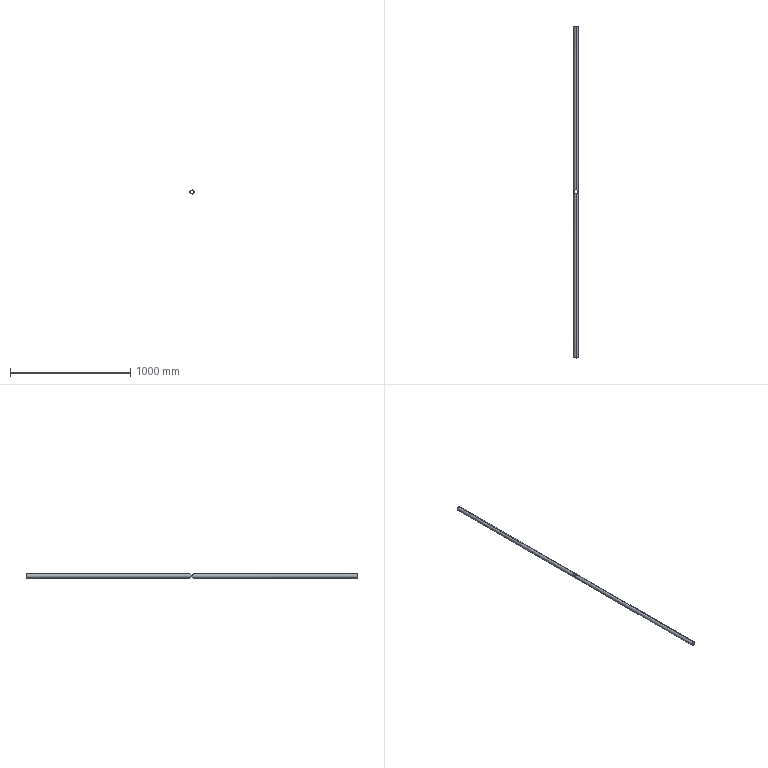Component | SolidWorks | PlatformGuardrail5-1 | 2 solids | 12 faces | box 33.5 x 2760 x 33.5 mm | volume 786282 mm3 | cylinder 10 | plane 2 | commonest cylinder face diameters 27.5 x4 33.5 x4 33.6 x2 | material Plain Carbon Steel
STEP:
#1=CARTESIAN_POINT('',(246.892,87.591,243.001));
#2=VERTEX_POINT('',#1);
#3=CARTESIAN_POINT('',(246.892,87.591,244.084));
#4=VERTEX_POINT('',#3);
#5=CARTESIAN_POINT('',(246.892,87.591,243.542));
#6=DIRECTION('',(0.,1.,0.));
#7=DIRECTION('',(0.,0.,1.));
#8=AXIS2_PLACEMENT_3D('',#5,#6,#7);
#9=CIRCLE('',#8,0.5413);
#10=EDGE_CURVE('',#2,#4,#9,.T.);
#11=ORIENTED_EDGE('',*,*,#10,.T.);
#12=CARTESIAN_POINT('',(246.892,34.05,244.084));
#13=VERTEX_POINT('',#12);
#14=CARTESIAN_POINT('',(246.892,87.591,244.084));
#15=DIRECTION('',(0.,-1.,0.));
#16=VECTOR('',#15,39.37);
#17=LINE('',#14,#16);
#18=EDGE_CURVE('',#4,#13,#17,.T.);
#19=ORIENTED_EDGE('',*,*,#18,.T.);
#20=CARTESIAN_POINT('',(246.892,34.05,243.001));
#21=VERTEX_POINT('',#20);
#22=CARTESIAN_POINT('',(246.892,34.05,243.001));
#23=CARTESIAN_POINT('',(246.854,34.05,243.001));
#24=CARTESIAN_POINT('',(246.816,34.047,243.005));
#25=CARTESIAN_POINT('',(246.762,34.038,243.016));
#26=CARTESIAN_POINT('',(246.744,34.034,243.021));
#27=CARTESIAN_POINT('',(246.709,34.025,243.032));
#28=CARTESIAN_POINT('',(246.692,34.019,243.039));
#29=CARTESIAN_POINT('',(246.659,34.008,243.053));
#30=CARTESIAN_POINT('',(246.643,34.002,243.061));
#31=CARTESIAN_POINT('',(246.612,33.988,243.078));
#32=CARTESIAN_POINT('',(246.597,33.981,243.088));
#33=CARTESIAN_POINT('',(246.555,33.959,243.117));
#34=CARTESIAN_POINT('',(246.529,33.942,243.139));
#35=CARTESIAN_POINT('',(246.494,33.917,243.175));
#36=CARTESIAN_POINT('',(246.482,33.908,243.188));
#37=CARTESIAN_POINT('',(246.461,33.891,243.214));
#38=CARTESIAN_POINT('',(246.451,33.882,243.227));
#39=CARTESIAN_POINT('',(246.423,33.856,243.269));
#40=CARTESIAN_POINT('',(246.407,33.839,243.298));
#41=CARTESIAN_POINT('',(246.387,33.816,243.346));
#42=CARTESIAN_POINT('',(246.381,33.809,243.362));
#43=CARTESIAN_POINT('',(246.37,33.796,243.396));
#44=CARTESIAN_POINT('',(246.366,33.79,243.413));
#45=CARTESIAN_POINT('',(246.358,33.78,243.449));
#46=CARTESIAN_POINT('',(246.355,33.776,243.467));
#47=CARTESIAN_POINT('',(246.351,33.77,243.505));
#48=CARTESIAN_POINT('',(246.35,33.769,243.524));
#49=CARTESIAN_POINT('',(246.35,33.769,243.561));
#50=CARTESIAN_POINT('',(246.351,33.77,243.58));
#51=CARTESIAN_POINT('',(246.354,33.774,243.608));
#52=CARTESIAN_POINT('',(246.356,33.776,243.617));
#53=CARTESIAN_POINT('',(246.358,33.78,243.636));
#54=CARTESIAN_POINT('',(246.36,33.782,243.645));
#55=CARTESIAN_POINT('',(246.366,33.79,243.671));
#56=CARTESIAN_POINT('',(246.37,33.796,243.689));
#57=CARTESIAN_POINT('',(246.381,33.809,243.722));
#58=CARTESIAN_POINT('',(246.387,33.816,243.739));
#59=CARTESIAN_POINT('',(246.407,33.84,243.787));
#60=CARTESIAN_POINT('',(246.423,33.857,243.816));
#61=CARTESIAN_POINT('',(246.451,33.882,243.858));
#62=CARTESIAN_POINT('',(246.461,33.891,243.871));
#63=CARTESIAN_POINT('',(246.483,33.908,243.897));
#64=CARTESIAN_POINT('',(246.494,33.917,243.91));
#65=CARTESIAN_POINT('',(246.529,33.943,243.946));
#66=CARTESIAN_POINT('',(246.555,33.959,243.967));
#67=CARTESIAN_POINT('',(246.597,33.981,243.997));
#68=CARTESIAN_POINT('',(246.612,33.988,244.006));
#69=CARTESIAN_POINT('',(246.643,34.002,244.023));
#70=CARTESIAN_POINT('',(246.659,34.008,244.031));
#71=CARTESIAN_POINT('',(246.692,34.02,244.046));
#72=CARTESIAN_POINT('',(246.709,34.025,244.052));
#73=CARTESIAN_POINT('',(246.744,34.034,244.063));
#74=CARTESIAN_POINT('',(246.762,34.037,244.068));
#75=CARTESIAN_POINT('',(246.817,34.047,244.08));
#76=CARTESIAN_POINT('',(246.854,34.05,244.084));
#77=CARTESIAN_POINT('',(246.892,34.05,244.084));
#78=B_SPLINE_CURVE_WITH_KNOTS('',3,(#22,#23,#24,#25,#26,#27,#28,#29,#30,#31,#32,#33,#34,#35,#36,#37,#38,#39,#40,#41,#42,#43,#44,#45,#46,#47,#48,#49,#50,#51,#52,#53,#54,#55,#56,#57,#58,#59,#60,#61,#62,#63,#64,#65,#66,#67,#68,#69,#70,#71,#72,#73,#74,#75,#76,#77),.UNSPECIFIED.,.F.,.F.,(4,2,2,2,2,2,2,2,2,2,2,2,2,2,2,2,2,2,2,2,2,2,2,2,2,2,2,4),(0.,0.002859,0.004288,0.005717,0.007146,0.008576,0.01143,0.01286,0.01429,0.01715,0.01858,0.02001,0.02144,0.02287,0.0243,0.02501,0.02573,0.02716,0.02859,0.03144,0.03287,0.0343,0.03716,0.03859,0.04002,0.04145,0.04288,0.04574),.UNSPECIFIED.);
#79=EDGE_CURVE('',#21,#13,#78,.T.);
#80=ORIENTED_EDGE('',*,*,#79,.F.);
#81=CARTESIAN_POINT('',(246.892,87.591,243.001));
#82=DIRECTION('',(0.,-1.,0.));
#83=VECTOR('',#82,39.37);
#84=LINE('',#81,#83);
#85=EDGE_CURVE('',#2,#21,#84,.T.);
#86=ORIENTED_EDGE('',*,*,#85,.F.);
#87=EDGE_LOOP('',(#11,#19,#80,#86));
#88=FACE_OUTER_BOUND('',#87,.T.);
#89=CARTESIAN_POINT('',(246.892,87.591,243.542));
#90=DIRECTION('',(0.,-1.,0.));
#91=DIRECTION('',(0.,0.,-1.));
#92=AXIS2_PLACEMENT_3D('',#89,#90,#91);
#93=CYLINDRICAL_SURFACE('',#92,0.5413);
#94=ADVANCED_FACE('',(#88),#93,.F.);
#95=CARTESIAN_POINT('',(246.892,87.591,244.202));
#96=VERTEX_POINT('',#95);
#97=CARTESIAN_POINT('',(246.892,87.591,242.883));
#98=VERTEX_POINT('',#97);
#99=CARTESIAN_POINT('',(246.892,87.591,243.542));
#100=DIRECTION('',(0.,1.,0.));
#101=DIRECTION('',(0.,0.,1.));
#102=AXIS2_PLACEMENT_3D('',#99,#100,#101);
#103=CIRCLE('',#102,0.6594);
#104=EDGE_CURVE('',#96,#98,#103,.T.);
#105=ORIENTED_EDGE('',*,*,#104,.F.);
#106=CARTESIAN_POINT('',(246.892,34.05,244.202));
#107=VERTEX_POINT('',#106);
#108=CARTESIAN_POINT('',(246.892,87.591,244.202));
#109=DIRECTION('',(0.,-1.,0.));
#110=VECTOR('',#109,39.37);
#111=LINE('',#108,#110);
#112=EDGE_CURVE('',#96,#107,#111,.T.);
#113=ORIENTED_EDGE('',*,*,#112,.T.);
#114=CARTESIAN_POINT('',(246.892,34.05,242.883));
#115=VERTEX_POINT('',#114);
#116=CARTESIAN_POINT('',(246.892,34.05,244.202));
#117=CARTESIAN_POINT('',(246.918,34.05,244.202));
#118=CARTESIAN_POINT('',(246.943,34.049,244.2));
#119=CARTESIAN_POINT('',(246.981,34.044,244.196));
#120=CARTESIAN_POINT('',(246.994,34.042,244.194));
#121=CARTESIAN_POINT('',(247.019,34.038,244.189));
#122=CARTESIAN_POINT('',(247.031,34.035,244.187));
#123=CARTESIAN_POINT('',(247.068,34.027,244.178));
#124=CARTESIAN_POINT('',(247.092,34.02,244.171));
#125=CARTESIAN_POINT('',(247.126,34.007,244.159));
#126=CARTESIAN_POINT('',(247.138,34.003,244.154));
#127=CARTESIAN_POINT('',(247.16,33.993,244.145));
#128=CARTESIAN_POINT('',(247.171,33.988,244.14));
#129=CARTESIAN_POINT('',(247.224,33.962,244.114));
#130=CARTESIAN_POINT('',(247.262,33.938,244.09));
#131=CARTESIAN_POINT('',(247.314,33.898,244.049));
#132=CARTESIAN_POINT('',(247.331,33.884,244.035));
#133=CARTESIAN_POINT('',(247.362,33.855,244.006));
#134=CARTESIAN_POINT('',(247.376,33.84,243.99));
#135=CARTESIAN_POINT('',(247.416,33.794,243.944));
#136=CARTESIAN_POINT('',(247.439,33.762,243.912));
#137=CARTESIAN_POINT('',(247.469,33.712,243.861));
#138=CARTESIAN_POINT('',(247.478,33.695,243.844));
#139=CARTESIAN_POINT('',(247.495,33.66,243.809));
#140=CARTESIAN_POINT('',(247.503,33.643,243.792));
#141=CARTESIAN_POINT('',(247.516,33.609,243.756));
#142=CARTESIAN_POINT('',(247.522,33.591,243.738));
#143=CARTESIAN_POINT('',(247.532,33.556,243.702));
#144=CARTESIAN_POINT('',(247.536,33.539,243.684));
#145=CARTESIAN_POINT('',(247.541,33.513,243.656));
#146=CARTESIAN_POINT('',(247.543,33.504,243.646));
#147=CARTESIAN_POINT('',(247.546,33.488,243.627));
#148=CARTESIAN_POINT('',(247.547,33.479,243.617));
#149=CARTESIAN_POINT('',(247.549,33.467,243.602));
#150=CARTESIAN_POINT('',(247.549,33.463,243.597));
#151=CARTESIAN_POINT('',(247.55,33.456,243.586));
#152=CARTESIAN_POINT('',(247.55,33.452,243.581));
#153=CARTESIAN_POINT('',(247.551,33.446,243.569));
#154=CARTESIAN_POINT('',(247.551,33.444,243.564));
#155=CARTESIAN_POINT('',(247.551,33.44,243.551));
#156=CARTESIAN_POINT('',(247.551,33.439,243.545));
#157=CARTESIAN_POINT('',(247.551,33.44,243.532));
#158=CARTESIAN_POINT('',(247.551,33.442,243.525));
#159=CARTESIAN_POINT('',(247.551,33.447,243.513));
#160=CARTESIAN_POINT('',(247.55,33.45,243.508));
#161=CARTESIAN_POINT('',(247.549,33.46,243.491));
#162=CARTESIAN_POINT('',(247.548,33.468,243.481));
#163=CARTESIAN_POINT('',(247.546,33.484,243.461));
#164=CARTESIAN_POINT('',(247.545,33.493,243.452));
#165=CARTESIAN_POINT('',(247.542,33.509,243.433));
#166=CARTESIAN_POINT('',(247.54,33.518,243.423));
#167=CARTESIAN_POINT('',(247.535,33.544,243.396));
#168=CARTESIAN_POINT('',(247.531,33.561,243.377));
#169=CARTESIAN_POINT('',(247.52,33.596,243.341));
#170=CARTESIAN_POINT('',(247.514,33.613,243.323));
#171=CARTESIAN_POINT('',(247.494,33.665,243.271));
#172=CARTESIAN_POINT('',(247.477,33.699,243.236));
#173=CARTESIAN_POINT('',(247.438,33.764,243.17));
#174=CARTESIAN_POINT('',(247.415,33.796,243.138));
#175=CARTESIAN_POINT('',(247.374,33.842,243.092));
#176=CARTESIAN_POINT('',(247.359,33.857,243.077));
#177=CARTESIAN_POINT('',(247.329,33.886,243.048));
#178=CARTESIAN_POINT('',(247.312,33.9,243.034));
#179=CARTESIAN_POINT('',(247.278,33.926,243.007));
#180=CARTESIAN_POINT('',(247.26,33.939,242.995));
#181=CARTESIAN_POINT('',(247.221,33.963,242.971));
#182=CARTESIAN_POINT('',(247.201,33.974,242.959));
#183=CARTESIAN_POINT('',(247.159,33.994,242.939));
#184=CARTESIAN_POINT('',(247.137,34.004,242.929));
#185=CARTESIAN_POINT('',(247.102,34.016,242.917));
#186=CARTESIAN_POINT('',(247.091,34.02,242.913));
#187=CARTESIAN_POINT('',(247.067,34.027,242.906));
#188=CARTESIAN_POINT('',(247.055,34.03,242.903));
#189=CARTESIAN_POINT('',(247.018,34.038,242.895));
#190=CARTESIAN_POINT('',(246.993,34.043,242.89));
#191=CARTESIAN_POINT('',(246.956,34.047,242.886));
#192=CARTESIAN_POINT('',(246.943,34.048,242.885));
#193=CARTESIAN_POINT('',(246.924,34.049,242.884));
#194=CARTESIAN_POINT('',(246.918,34.05,242.883));
#195=CARTESIAN_POINT('',(246.905,34.05,242.883));
#196=CARTESIAN_POINT('',(246.898,34.05,242.883));
#197=CARTESIAN_POINT('',(246.892,34.05,242.883));
#198=B_SPLINE_CURVE_WITH_KNOTS('',3,(#116,#117,#118,#119,#120,#121,#122,#123,#124,#125,#126,#127,#128,#129,#130,#131,#132,#133,#134,#135,#136,#137,#138,#139,#140,#141,#142,#143,#144,#145,#146,#147,#148,#149,#150,#151,#152,#153,#154,#155,#156,#157,#158,#159,#160,#161,#162,#163,#164,#165,#166,#167,#168,#169,#170,#171,#172,#173,#174,#175,#176,#177,#178,#179,#180,#181,#182,#183,#184,#185,#186,#187,#188,#189,#190,#191,#192,#193,#194,#195,#196,#197),.UNSPECIFIED.,.F.,.F.,(4,2,2,2,2,2,2,2,2,2,2,2,2,2,2,2,2,2,2,2,2,2,2,2,2,2,2,2,2,2,2,2,2,2,2,2,2,2,2,2,4),(0.06181,0.06373,0.0647,0.06566,0.06759,0.06855,0.06951,0.07337,0.07529,0.07722,0.08107,0.083,0.08492,0.08685,0.08878,0.08974,0.0907,0.09118,0.09167,0.09215,0.09263,0.09311,0.09359,0.09456,0.09552,0.09648,0.09841,0.1003,0.1042,0.108,0.11,0.1119,0.1138,0.1157,0.1177,0.1186,0.1196,0.1215,0.1225,0.123,0.1235),.UNSPECIFIED.);
#199=EDGE_CURVE('',#107,#115,#198,.T.);
#200=ORIENTED_EDGE('',*,*,#199,.T.);
#201=CARTESIAN_POINT('',(246.892,87.591,242.883));
#202=DIRECTION('',(0.,-1.,0.));
#203=VECTOR('',#202,39.37);
#204=LINE('',#201,#203);
#205=EDGE_CURVE('',#98,#115,#204,.T.);
#206=ORIENTED_EDGE('',*,*,#205,.F.);
#207=EDGE_LOOP('',(#105,#113,#200,#206));
#208=FACE_OUTER_BOUND('',#207,.T.);
#209=CARTESIAN_POINT('',(246.892,87.591,243.542));
#210=DIRECTION('',(0.,-1.,0.));
#211=DIRECTION('',(0.,0.,-1.));
#212=AXIS2_PLACEMENT_3D('',#209,#210,#211);
#213=CYLINDRICAL_SURFACE('',#212,0.6594);
#214=ADVANCED_FACE('',(#208),#213,.T.);
#215=ORIENTED_EDGE('',*,*,#112,.F.);
#216=CARTESIAN_POINT('',(246.892,87.591,243.542));
#217=DIRECTION('',(0.,1.,0.));
#218=DIRECTION('',(0.,0.,1.));
#219=AXIS2_PLACEMENT_3D('',#216,#217,#218);
#220=CIRCLE('',#219,0.6594);
#221=EDGE_CURVE('',#98,#96,#220,.T.);
#222=ORIENTED_EDGE('',*,*,#221,.F.);
#223=ORIENTED_EDGE('',*,*,#205,.T.);
#224=CARTESIAN_POINT('',(246.892,34.05,242.883));
#225=CARTESIAN_POINT('',(246.84,34.05,242.883));
#226=CARTESIAN_POINT('',(246.79,34.044,242.889));
#227=CARTESIAN_POINT('',(246.729,34.03,242.903));
#228=CARTESIAN_POINT('',(246.717,34.027,242.906));
#229=CARTESIAN_POINT('',(246.694,34.02,242.913));
#230=CARTESIAN_POINT('',(246.682,34.016,242.917));
#231=CARTESIAN_POINT('',(246.648,34.004,242.929));
#232=CARTESIAN_POINT('',(246.626,33.995,242.938));
#233=CARTESIAN_POINT('',(246.584,33.975,242.959));
#234=CARTESIAN_POINT('',(246.563,33.963,242.97));
#235=CARTESIAN_POINT('',(246.525,33.94,242.994));
#236=CARTESIAN_POINT('',(246.507,33.927,243.006));
#237=CARTESIAN_POINT('',(246.473,33.901,243.033));
#238=CARTESIAN_POINT('',(246.456,33.887,243.047));
#239=CARTESIAN_POINT('',(246.426,33.858,243.075));
#240=CARTESIAN_POINT('',(246.411,33.844,243.09));
#241=CARTESIAN_POINT('',(246.37,33.798,243.136));
#242=CARTESIAN_POINT('',(246.347,33.766,243.168));
#243=CARTESIAN_POINT('',(246.307,33.701,243.234));
#244=CARTESIAN_POINT('',(246.291,33.667,243.268));
#245=CARTESIAN_POINT('',(246.27,33.616,243.321));
#246=CARTESIAN_POINT('',(246.264,33.598,243.339));
#247=CARTESIAN_POINT('',(246.254,33.564,243.375));
#248=CARTESIAN_POINT('',(246.249,33.546,243.393));
#249=CARTESIAN_POINT('',(246.243,33.52,243.421));
#250=CARTESIAN_POINT('',(246.242,33.512,243.43));
#251=CARTESIAN_POINT('',(246.239,33.495,243.449));
#252=CARTESIAN_POINT('',(246.238,33.486,243.459));
#253=CARTESIAN_POINT('',(246.235,33.47,243.478));
#254=CARTESIAN_POINT('',(246.234,33.462,243.488));
#255=CARTESIAN_POINT('',(246.233,33.452,243.504));
#256=CARTESIAN_POINT('',(246.233,33.449,243.51));
#257=CARTESIAN_POINT('',(246.233,33.443,243.522));
#258=CARTESIAN_POINT('',(246.232,33.441,243.528));
#259=CARTESIAN_POINT('',(246.232,33.439,243.541));
#260=CARTESIAN_POINT('',(246.232,33.44,243.547));
#261=CARTESIAN_POINT('',(246.233,33.442,243.56));
#262=CARTESIAN_POINT('',(246.233,33.445,243.566));
#263=CARTESIAN_POINT('',(246.234,33.454,243.584));
#264=CARTESIAN_POINT('',(246.234,33.461,243.594));
#265=CARTESIAN_POINT('',(246.236,33.477,243.615));
#266=CARTESIAN_POINT('',(246.237,33.485,243.624));
#267=CARTESIAN_POINT('',(246.24,33.502,243.644));
#268=CARTESIAN_POINT('',(246.242,33.511,243.653));
#269=CARTESIAN_POINT('',(246.247,33.537,243.682));
#270=CARTESIAN_POINT('',(246.251,33.554,243.7));
#271=CARTESIAN_POINT('',(246.261,33.59,243.737));
#272=CARTESIAN_POINT('',(246.267,33.607,243.755));
#273=CARTESIAN_POINT('',(246.287,33.659,243.808));
#274=CARTESIAN_POINT('',(246.303,33.693,243.843));
#275=CARTESIAN_POINT('',(246.333,33.743,243.893));
#276=CARTESIAN_POINT('',(246.344,33.76,243.91));
#277=CARTESIAN_POINT('',(246.367,33.792,243.942));
#278=CARTESIAN_POINT('',(246.38,33.808,243.958));
#279=CARTESIAN_POINT('',(246.42,33.854,244.005));
#280=CARTESIAN_POINT('',(246.451,33.884,244.035));
#281=CARTESIAN_POINT('',(246.503,33.924,244.075));
#282=CARTESIAN_POINT('',(246.521,33.937,244.088));
#283=CARTESIAN_POINT('',(246.56,33.961,244.113));
#284=CARTESIAN_POINT('',(246.58,33.973,244.124));
#285=CARTESIAN_POINT('',(246.623,33.993,244.145));
#286=CARTESIAN_POINT('',(246.645,34.003,244.154));
#287=CARTESIAN_POINT('',(246.691,34.019,244.171));
#288=CARTESIAN_POINT('',(246.715,34.027,244.178));
#289=CARTESIAN_POINT('',(246.764,34.038,244.19));
#290=CARTESIAN_POINT('',(246.789,34.043,244.194));
#291=CARTESIAN_POINT('',(246.84,34.049,244.2));
#292=CARTESIAN_POINT('',(246.866,34.05,244.202));
#293=CARTESIAN_POINT('',(246.892,34.05,244.202));
#294=B_SPLINE_CURVE_WITH_KNOTS('',3,(#224,#225,#226,#227,#228,#229,#230,#231,#232,#233,#234,#235,#236,#237,#238,#239,#240,#241,#242,#243,#244,#245,#246,#247,#248,#249,#250,#251,#252,#253,#254,#255,#256,#257,#258,#259,#260,#261,#262,#263,#264,#265,#266,#267,#268,#269,#270,#271,#272,#273,#274,#275,#276,#277,#278,#279,#280,#281,#282,#283,#284,#285,#286,#287,#288,#289,#290,#291,#292,#293),.UNSPECIFIED.,.F.,.F.,(4,2,2,2,2,2,2,2,2,2,2,2,2,2,2,2,2,2,2,2,2,2,2,2,2,2,2,2,2,2,2,2,2,2,4),(0.,0.003863,0.004829,0.005795,0.007726,0.009658,0.01159,0.01352,0.01545,0.01932,0.02318,0.02511,0.02704,0.02801,0.02897,0.02994,0.03042,0.0309,0.03139,0.03187,0.03284,0.0338,0.03477,0.0367,0.03863,0.04249,0.04442,0.04636,0.05022,0.05215,0.05408,0.05601,0.05795,0.05988,0.06181),.UNSPECIFIED.);
#295=EDGE_CURVE('',#115,#107,#294,.T.);
#296=ORIENTED_EDGE('',*,*,#295,.T.);
#297=EDGE_LOOP('',(#215,#222,#223,#296));
#298=FACE_OUTER_BOUND('',#297,.T.);
#299=CARTESIAN_POINT('',(246.892,87.591,243.542));
#300=DIRECTION('',(0.,-1.,0.));
#301=DIRECTION('',(0.,0.,-1.));
#302=AXIS2_PLACEMENT_3D('',#299,#300,#301);
#303=CYLINDRICAL_SURFACE('',#302,0.6594);
#304=ADVANCED_FACE('',(#298),#303,.T.);
#305=ORIENTED_EDGE('',*,*,#18,.F.);
#306=CARTESIAN_POINT('',(246.892,87.591,243.542));
#307=DIRECTION('',(0.,1.,0.));
#308=DIRECTION('',(0.,0.,1.));
#309=AXIS2_PLACEMENT_3D('',#306,#307,#308);
#310=CIRCLE('',#309,0.5413);
#311=EDGE_CURVE('',#4,#2,#310,.T.);
#312=ORIENTED_EDGE('',*,*,#311,.T.);
#313=ORIENTED_EDGE('',*,*,#85,.T.);
#314=CARTESIAN_POINT('',(246.892,34.05,244.084));
#315=CARTESIAN_POINT('',(246.901,34.05,244.084));
#316=CARTESIAN_POINT('',(246.911,34.05,244.083));
#317=CARTESIAN_POINT('',(246.929,34.049,244.082));
#318=CARTESIAN_POINT('',(246.939,34.048,244.082));
#319=CARTESIAN_POINT('',(246.967,34.046,244.079));
#320=CARTESIAN_POINT('',(246.986,34.044,244.076));
#321=CARTESIAN_POINT('',(247.022,34.037,244.068));
#322=CARTESIAN_POINT('',(247.04,34.034,244.063));
#323=CARTESIAN_POINT('',(247.075,34.025,244.052));
#324=CARTESIAN_POINT('',(247.092,34.019,244.046));
#325=CARTESIAN_POINT('',(247.125,34.008,244.031));
#326=CARTESIAN_POINT('',(247.141,34.002,244.023));
#327=CARTESIAN_POINT('',(247.171,33.988,244.006));
#328=CARTESIAN_POINT('',(247.186,33.981,243.997));
#329=CARTESIAN_POINT('',(247.229,33.959,243.967));
#330=CARTESIAN_POINT('',(247.255,33.942,243.945));
#331=CARTESIAN_POINT('',(247.29,33.917,243.909));
#332=CARTESIAN_POINT('',(247.301,33.908,243.897));
#333=CARTESIAN_POINT('',(247.322,33.891,243.871));
#334=CARTESIAN_POINT('',(247.332,33.882,243.858));
#335=CARTESIAN_POINT('',(247.36,33.856,243.816));
#336=CARTESIAN_POINT('',(247.376,33.84,243.786));
#337=CARTESIAN_POINT('',(247.396,33.817,243.739));
#338=CARTESIAN_POINT('',(247.402,33.809,243.723));
#339=CARTESIAN_POINT('',(247.413,33.796,243.69));
#340=CARTESIAN_POINT('',(247.418,33.79,243.672));
#341=CARTESIAN_POINT('',(247.425,33.78,243.636));
#342=CARTESIAN_POINT('',(247.428,33.776,243.618));
#343=CARTESIAN_POINT('',(247.431,33.772,243.59));
#344=CARTESIAN_POINT('',(247.432,33.771,243.581));
#345=CARTESIAN_POINT('',(247.433,33.769,243.562));
#346=CARTESIAN_POINT('',(247.433,33.769,243.552));
#347=CARTESIAN_POINT('',(247.433,33.769,243.524));
#348=CARTESIAN_POINT('',(247.432,33.77,243.505));
#349=CARTESIAN_POINT('',(247.428,33.775,243.468));
#350=CARTESIAN_POINT('',(247.425,33.78,243.45));
#351=CARTESIAN_POINT('',(247.414,33.795,243.396));
#352=CARTESIAN_POINT('',(247.404,33.808,243.362));
#353=CARTESIAN_POINT('',(247.383,33.831,243.315));
#354=CARTESIAN_POINT('',(247.376,33.84,243.299));
#355=CARTESIAN_POINT('',(247.36,33.856,243.269));
#356=CARTESIAN_POINT('',(247.351,33.865,243.255));
#357=CARTESIAN_POINT('',(247.323,33.891,243.214));
#358=CARTESIAN_POINT('',(247.302,33.908,243.188));
#359=CARTESIAN_POINT('',(247.267,33.934,243.151));
#360=CARTESIAN_POINT('',(247.254,33.942,243.14));
#361=CARTESIAN_POINT('',(247.228,33.958,243.118));
#362=CARTESIAN_POINT('',(247.215,33.966,243.108));
#363=CARTESIAN_POINT('',(247.173,33.988,243.078));
#364=CARTESIAN_POINT('',(247.142,34.002,243.061));
#365=CARTESIAN_POINT('',(247.093,34.019,243.039));
#366=CARTESIAN_POINT('',(247.075,34.024,243.033));
#367=CARTESIAN_POINT('',(247.041,34.033,243.021));
#368=CARTESIAN_POINT('',(247.023,34.037,243.017));
#369=CARTESIAN_POINT('',(246.986,34.044,243.009));
#370=CARTESIAN_POINT('',(246.968,34.046,243.006));
#371=CARTESIAN_POINT('',(246.93,34.049,243.002));
#372=CARTESIAN_POINT('',(246.911,34.05,243.001));
#373=CARTESIAN_POINT('',(246.892,34.05,243.001));
#374=B_SPLINE_CURVE_WITH_KNOTS('',3,(#314,#315,#316,#317,#318,#319,#320,#321,#322,#323,#324,#325,#326,#327,#328,#329,#330,#331,#332,#333,#334,#335,#336,#337,#338,#339,#340,#341,#342,#343,#344,#345,#346,#347,#348,#349,#350,#351,#352,#353,#354,#355,#356,#357,#358,#359,#360,#361,#362,#363,#364,#365,#366,#367,#368,#369,#370,#371,#372,#373),.UNSPECIFIED.,.F.,.F.,(4,2,2,2,2,2,2,2,2,2,2,2,2,2,2,2,2,2,2,2,2,2,2,2,2,2,2,2,2,4),(0.04574,0.04645,0.04716,0.04859,0.05001,0.05144,0.05286,0.05429,0.05714,0.05857,0.05999,0.06284,0.06427,0.0657,0.06712,0.06783,0.06855,0.06997,0.0714,0.07425,0.07568,0.0771,0.07995,0.08138,0.0828,0.08566,0.08708,0.08851,0.08993,0.09136),.UNSPECIFIED.);
#375=EDGE_CURVE('',#13,#21,#374,.T.);
#376=ORIENTED_EDGE('',*,*,#375,.F.);
#377=EDGE_LOOP('',(#305,#312,#313,#376));
#378=FACE_OUTER_BOUND('',#377,.T.);
#379=CARTESIAN_POINT('',(246.892,87.591,243.542));
#380=DIRECTION('',(0.,-1.,0.));
#381=DIRECTION('',(0.,0.,-1.));
#382=AXIS2_PLACEMENT_3D('',#379,#380,#381);
#383=CYLINDRICAL_SURFACE('',#382,0.5413);
#384=ADVANCED_FACE('',(#378),#383,.F.);
#385=ORIENTED_EDGE('',*,*,#221,.T.);
#386=ORIENTED_EDGE('',*,*,#104,.T.);
#387=EDGE_LOOP('',(#385,#386));
#388=FACE_OUTER_BOUND('',#387,.T.);
#389=ORIENTED_EDGE('',*,*,#10,.F.);
#390=ORIENTED_EDGE('',*,*,#311,.F.);
#391=EDGE_LOOP('',(#389,#390));
#392=FACE_BOUND('',#391,.T.);
#393=CARTESIAN_POINT('',(246.892,87.591,243.542));
#394=DIRECTION('',(0.,1.,0.));
#395=DIRECTION('',(0.,0.,1.));
#396=AXIS2_PLACEMENT_3D('',#393,#394,#395);
#397=PLANE('',#396);
#398=ADVANCED_FACE('',(#388,#392),#397,.T.);
#399=ORIENTED_EDGE('',*,*,#79,.T.);
#400=ORIENTED_EDGE('',*,*,#375,.T.);
#401=EDGE_LOOP('',(#399,#400));
#402=FACE_BOUND('',#401,.T.);
#403=ORIENTED_EDGE('',*,*,#295,.F.);
#404=ORIENTED_EDGE('',*,*,#199,.F.);
#405=EDGE_LOOP('',(#403,#404));
#406=FACE_OUTER_BOUND('',#405,.T.);
#407=CARTESIAN_POINT('',(246.892,33.389,242.883));
#408=DIRECTION('',(0.,0.,1.));
#409=DIRECTION('',(1.,0.,0.));
#410=AXIS2_PLACEMENT_3D('',#407,#408,#409);
#411=CYLINDRICAL_SURFACE('',#410,0.6614);
#412=ADVANCED_FACE('',(#402,#406),#411,.F.);
#413=CLOSED_SHELL('',(#94,#214,#304,#384,#398,#412));
#414=MANIFOLD_SOLID_BREP('',#413);
#415=CARTESIAN_POINT('',(246.892,32.727,244.084));
#416=VERTEX_POINT('',#415);
#417=CARTESIAN_POINT('',(246.892,32.727,243.001));
#418=VERTEX_POINT('',#417);
#419=CARTESIAN_POINT('',(246.892,32.727,244.084));
#420=CARTESIAN_POINT('',(246.882,32.727,244.084));
#421=CARTESIAN_POINT('',(246.873,32.727,244.083));
#422=CARTESIAN_POINT('',(246.854,32.728,244.082));
#423=CARTESIAN_POINT('',(246.845,32.729,244.082));
#424=CARTESIAN_POINT('',(246.816,32.731,244.079));
#425=CARTESIAN_POINT('',(246.798,32.734,244.076));
#426=CARTESIAN_POINT('',(246.762,32.74,244.068));
#427=CARTESIAN_POINT('',(246.744,32.744,244.063));
#428=CARTESIAN_POINT('',(246.709,32.753,244.052));
#429=CARTESIAN_POINT('',(246.692,32.758,244.046));
#430=CARTESIAN_POINT('',(246.659,32.769,244.031));
#431=CARTESIAN_POINT('',(246.643,32.776,244.023));
#432=CARTESIAN_POINT('',(246.612,32.789,244.006));
#433=CARTESIAN_POINT('',(246.597,32.796,243.997));
#434=CARTESIAN_POINT('',(246.554,32.819,243.967));
#435=CARTESIAN_POINT('',(246.529,32.835,243.945));
#436=CARTESIAN_POINT('',(246.494,32.86,243.909));
#437=CARTESIAN_POINT('',(246.483,32.869,243.897));
#438=CARTESIAN_POINT('',(246.461,32.886,243.871));
#439=CARTESIAN_POINT('',(246.451,32.895,243.858));
#440=CARTESIAN_POINT('',(246.423,32.921,243.816));
#441=CARTESIAN_POINT('',(246.407,32.938,243.786));
#442=CARTESIAN_POINT('',(246.387,32.961,243.739));
#443=CARTESIAN_POINT('',(246.381,32.968,243.723));
#444=CARTESIAN_POINT('',(246.371,32.981,243.69));
#445=CARTESIAN_POINT('',(246.366,32.987,243.672));
#446=CARTESIAN_POINT('',(246.358,32.998,243.636));
#447=CARTESIAN_POINT('',(246.355,33.002,243.618));
#448=CARTESIAN_POINT('',(246.352,33.006,243.59));
#449=CARTESIAN_POINT('',(246.352,33.007,243.581));
#450=CARTESIAN_POINT('',(246.351,33.008,243.562));
#451=CARTESIAN_POINT('',(246.35,33.009,243.552));
#452=CARTESIAN_POINT('',(246.35,33.009,243.524));
#453=CARTESIAN_POINT('',(246.351,33.007,243.505));
#454=CARTESIAN_POINT('',(246.355,33.002,243.468));
#455=CARTESIAN_POINT('',(246.358,32.998,243.45));
#456=CARTESIAN_POINT('',(246.369,32.983,243.396));
#457=CARTESIAN_POINT('',(246.38,32.969,243.362));
#458=CARTESIAN_POINT('',(246.4,32.946,243.315));
#459=CARTESIAN_POINT('',(246.408,32.938,243.299));
#460=CARTESIAN_POINT('',(246.424,32.921,243.269));
#461=CARTESIAN_POINT('',(246.433,32.913,243.255));
#462=CARTESIAN_POINT('',(246.46,32.887,243.214));
#463=CARTESIAN_POINT('',(246.481,32.869,243.188));
#464=CARTESIAN_POINT('',(246.517,32.844,243.151));
#465=CARTESIAN_POINT('',(246.529,32.835,243.14));
#466=CARTESIAN_POINT('',(246.555,32.819,243.118));
#467=CARTESIAN_POINT('',(246.569,32.811,243.108));
#468=CARTESIAN_POINT('',(246.611,32.789,243.078));
#469=CARTESIAN_POINT('',(246.641,32.776,243.061));
#470=CARTESIAN_POINT('',(246.691,32.758,243.039));
#471=CARTESIAN_POINT('',(246.708,32.753,243.033));
#472=CARTESIAN_POINT('',(246.743,32.744,243.021));
#473=CARTESIAN_POINT('',(246.761,32.74,243.017));
#474=CARTESIAN_POINT('',(246.797,32.734,243.009));
#475=CARTESIAN_POINT('',(246.816,32.731,243.006));
#476=CARTESIAN_POINT('',(246.854,32.728,243.002));
#477=CARTESIAN_POINT('',(246.873,32.727,243.001));
#478=CARTESIAN_POINT('',(246.892,32.727,243.001));
#479=B_SPLINE_CURVE_WITH_KNOTS('',3,(#419,#420,#421,#422,#423,#424,#425,#426,#427,#428,#429,#430,#431,#432,#433,#434,#435,#436,#437,#438,#439,#440,#441,#442,#443,#444,#445,#446,#447,#448,#449,#450,#451,#452,#453,#454,#455,#456,#457,#458,#459,#460,#461,#462,#463,#464,#465,#466,#467,#468,#469,#470,#471,#472,#473,#474,#475,#476,#477,#478),.UNSPECIFIED.,.F.,.F.,(4,2,2,2,2,2,2,2,2,2,2,2,2,2,2,2,2,2,2,2,2,2,2,2,2,2,2,2,2,4),(0.04574,0.04645,0.04716,0.04859,0.05001,0.05144,0.05286,0.05429,0.05714,0.05857,0.05999,0.06284,0.06427,0.0657,0.06712,0.06783,0.06855,0.06997,0.0714,0.07425,0.07568,0.0771,0.07995,0.08138,0.0828,0.08566,0.08708,0.08851,0.08993,0.09136),.UNSPECIFIED.);
#480=EDGE_CURVE('',#416,#418,#479,.T.);
#481=ORIENTED_EDGE('',*,*,#480,.F.);
#482=CARTESIAN_POINT('',(246.892,-21.07,244.084));
#483=VERTEX_POINT('',#482);
#484=CARTESIAN_POINT('',(246.892,87.591,244.084));
#485=DIRECTION('',(0.,-1.,0.));
#486=VECTOR('',#485,39.37);
#487=LINE('',#484,#486);
#488=EDGE_CURVE('',#416,#483,#487,.T.);
#489=ORIENTED_EDGE('',*,*,#488,.T.);
#490=CARTESIAN_POINT('',(246.892,-21.07,243.001));
#491=VERTEX_POINT('',#490);
#492=CARTESIAN_POINT('',(246.892,-21.07,243.542));
#493=DIRECTION('',(0.,1.,0.));
#494=DIRECTION('',(0.,0.,1.));
#495=AXIS2_PLACEMENT_3D('',#492,#493,#494);
#496=CIRCLE('',#495,0.5413);
#497=EDGE_CURVE('',#491,#483,#496,.T.);
#498=ORIENTED_EDGE('',*,*,#497,.F.);
#499=CARTESIAN_POINT('',(246.892,87.591,243.001));
#500=DIRECTION('',(0.,-1.,0.));
#501=VECTOR('',#500,39.37);
#502=LINE('',#499,#501);
#503=EDGE_CURVE('',#418,#491,#502,.T.);
#504=ORIENTED_EDGE('',*,*,#503,.F.);
#505=EDGE_LOOP('',(#481,#489,#498,#504));
#506=FACE_OUTER_BOUND('',#505,.T.);
#507=CARTESIAN_POINT('',(246.892,87.591,243.542));
#508=DIRECTION('',(0.,-1.,0.));
#509=DIRECTION('',(0.,0.,-1.));
#510=AXIS2_PLACEMENT_3D('',#507,#508,#509);
#511=CYLINDRICAL_SURFACE('',#510,0.5413);
#512=ADVANCED_FACE('',(#506),#511,.F.);
#513=CARTESIAN_POINT('',(246.892,32.727,242.883));
#514=VERTEX_POINT('',#513);
#515=CARTESIAN_POINT('',(246.892,32.727,244.202));
#516=VERTEX_POINT('',#515);
#517=CARTESIAN_POINT('',(246.892,32.727,242.883));
#518=CARTESIAN_POINT('',(246.943,32.727,242.883));
#519=CARTESIAN_POINT('',(246.993,32.733,242.889));
#520=CARTESIAN_POINT('',(247.054,32.747,242.903));
#521=CARTESIAN_POINT('',(247.066,32.751,242.906));
#522=CARTESIAN_POINT('',(247.09,32.758,242.913));
#523=CARTESIAN_POINT('',(247.101,32.761,242.917));
#524=CARTESIAN_POINT('',(247.136,32.773,242.929));
#525=CARTESIAN_POINT('',(247.157,32.783,242.938));
#526=CARTESIAN_POINT('',(247.2,32.803,242.959));
#527=CARTESIAN_POINT('',(247.22,32.814,242.97));
#528=CARTESIAN_POINT('',(247.258,32.838,242.994));
#529=CARTESIAN_POINT('',(247.277,32.85,243.006));
#530=CARTESIAN_POINT('',(247.311,32.877,243.033));
#531=CARTESIAN_POINT('',(247.327,32.89,243.047));
#532=CARTESIAN_POINT('',(247.358,32.919,243.075));
#533=CARTESIAN_POINT('',(247.372,32.934,243.09));
#534=CARTESIAN_POINT('',(247.413,32.98,243.136));
#535=CARTESIAN_POINT('',(247.436,33.011,243.168));
#536=CARTESIAN_POINT('',(247.476,33.077,243.234));
#537=CARTESIAN_POINT('',(247.493,33.11,243.268));
#538=CARTESIAN_POINT('',(247.513,33.162,243.321));
#539=CARTESIAN_POINT('',(247.519,33.179,243.339));
#540=CARTESIAN_POINT('',(247.53,33.214,243.375));
#541=CARTESIAN_POINT('',(247.534,33.231,243.393));
#542=CARTESIAN_POINT('',(247.54,33.257,243.421));
#543=CARTESIAN_POINT('',(247.542,33.266,243.43));
#544=CARTESIAN_POINT('',(247.545,33.283,243.449));
#545=CARTESIAN_POINT('',(247.546,33.291,243.459));
#546=CARTESIAN_POINT('',(247.548,33.307,243.478));
#547=CARTESIAN_POINT('',(247.549,33.315,243.488));
#548=CARTESIAN_POINT('',(247.55,33.325,243.504));
#549=CARTESIAN_POINT('',(247.55,33.329,243.51));
#550=CARTESIAN_POINT('',(247.551,33.334,243.522));
#551=CARTESIAN_POINT('',(247.551,33.336,243.528));
#552=CARTESIAN_POINT('',(247.551,33.338,243.541));
#553=CARTESIAN_POINT('',(247.551,33.338,243.547));
#554=CARTESIAN_POINT('',(247.551,33.335,243.56));
#555=CARTESIAN_POINT('',(247.551,33.333,243.566));
#556=CARTESIAN_POINT('',(247.55,33.324,243.584));
#557=CARTESIAN_POINT('',(247.549,33.316,243.594));
#558=CARTESIAN_POINT('',(247.547,33.3,243.615));
#559=CARTESIAN_POINT('',(247.546,33.292,243.624));
#560=CARTESIAN_POINT('',(247.543,33.275,243.644));
#561=CARTESIAN_POINT('',(247.542,33.267,243.653));
#562=CARTESIAN_POINT('',(247.537,33.241,243.682));
#563=CARTESIAN_POINT('',(247.532,33.223,243.7));
#564=CARTESIAN_POINT('',(247.522,33.188,243.737));
#565=CARTESIAN_POINT('',(247.516,33.17,243.755));
#566=CARTESIAN_POINT('',(247.496,33.118,243.808));
#567=CARTESIAN_POINT('',(247.48,33.084,243.843));
#568=CARTESIAN_POINT('',(247.451,33.034,243.893));
#569=CARTESIAN_POINT('',(247.44,33.018,243.91));
#570=CARTESIAN_POINT('',(247.416,32.986,243.942));
#571=CARTESIAN_POINT('',(247.404,32.97,243.958));
#572=CARTESIAN_POINT('',(247.363,32.923,244.005));
#573=CARTESIAN_POINT('',(247.333,32.894,244.035));
#574=CARTESIAN_POINT('',(247.281,32.853,244.075));
#575=CARTESIAN_POINT('',(247.262,32.84,244.088));
#576=CARTESIAN_POINT('',(247.224,32.816,244.113));
#577=CARTESIAN_POINT('',(247.203,32.805,244.124));
#578=CARTESIAN_POINT('',(247.161,32.784,244.145));
#579=CARTESIAN_POINT('',(247.139,32.775,244.154));
#580=CARTESIAN_POINT('',(247.093,32.758,244.171));
#581=CARTESIAN_POINT('',(247.069,32.751,244.178));
#582=CARTESIAN_POINT('',(247.02,32.739,244.19));
#583=CARTESIAN_POINT('',(246.995,32.735,244.194));
#584=CARTESIAN_POINT('',(246.944,32.729,244.2));
#585=CARTESIAN_POINT('',(246.918,32.727,244.202));
#586=CARTESIAN_POINT('',(246.892,32.727,244.202));
#587=B_SPLINE_CURVE_WITH_KNOTS('',3,(#517,#518,#519,#520,#521,#522,#523,#524,#525,#526,#527,#528,#529,#530,#531,#532,#533,#534,#535,#536,#537,#538,#539,#540,#541,#542,#543,#544,#545,#546,#547,#548,#549,#550,#551,#552,#553,#554,#555,#556,#557,#558,#559,#560,#561,#562,#563,#564,#565,#566,#567,#568,#569,#570,#571,#572,#573,#574,#575,#576,#577,#578,#579,#580,#581,#582,#583,#584,#585,#586),.UNSPECIFIED.,.F.,.F.,(4,2,2,2,2,2,2,2,2,2,2,2,2,2,2,2,2,2,2,2,2,2,2,2,2,2,2,2,2,2,2,2,2,2,4),(0.,0.003863,0.004829,0.005795,0.007726,0.009658,0.01159,0.01352,0.01545,0.01932,0.02318,0.02511,0.02704,0.02801,0.02897,0.02994,0.03042,0.0309,0.03139,0.03187,0.03284,0.0338,0.03477,0.0367,0.03863,0.04249,0.04442,0.04636,0.05022,0.05215,0.05408,0.05601,0.05795,0.05988,0.06181),.UNSPECIFIED.);
#588=EDGE_CURVE('',#514,#516,#587,.T.);
#589=ORIENTED_EDGE('',*,*,#588,.T.);
#590=CARTESIAN_POINT('',(246.892,-21.07,244.202));
#591=VERTEX_POINT('',#590);
#592=CARTESIAN_POINT('',(246.892,87.591,244.202));
#593=DIRECTION('',(0.,-1.,0.));
#594=VECTOR('',#593,39.37);
#595=LINE('',#592,#594);
#596=EDGE_CURVE('',#516,#591,#595,.T.);
#597=ORIENTED_EDGE('',*,*,#596,.T.);
#598=CARTESIAN_POINT('',(246.892,-21.07,242.883));
#599=VERTEX_POINT('',#598);
#600=CARTESIAN_POINT('',(246.892,-21.07,243.542));
#601=DIRECTION('',(0.,1.,0.));
#602=DIRECTION('',(0.,0.,1.));
#603=AXIS2_PLACEMENT_3D('',#600,#601,#602);
#604=CIRCLE('',#603,0.6594);
#605=EDGE_CURVE('',#591,#599,#604,.T.);
#606=ORIENTED_EDGE('',*,*,#605,.T.);
#607=CARTESIAN_POINT('',(246.892,87.591,242.883));
#608=DIRECTION('',(0.,-1.,0.));
#609=VECTOR('',#608,39.37);
#610=LINE('',#607,#609);
#611=EDGE_CURVE('',#514,#599,#610,.T.);
#612=ORIENTED_EDGE('',*,*,#611,.F.);
#613=EDGE_LOOP('',(#589,#597,#606,#612));
#614=FACE_OUTER_BOUND('',#613,.T.);
#615=CARTESIAN_POINT('',(246.892,87.591,243.542));
#616=DIRECTION('',(0.,-1.,0.));
#617=DIRECTION('',(0.,0.,-1.));
#618=AXIS2_PLACEMENT_3D('',#615,#616,#617);
#619=CYLINDRICAL_SURFACE('',#618,0.6594);
#620=ADVANCED_FACE('',(#614),#619,.T.);
#621=ORIENTED_EDGE('',*,*,#596,.F.);
#622=CARTESIAN_POINT('',(246.892,32.727,244.202));
#623=CARTESIAN_POINT('',(246.866,32.727,244.202));
#624=CARTESIAN_POINT('',(246.84,32.729,244.2));
#625=CARTESIAN_POINT('',(246.802,32.733,244.196));
#626=CARTESIAN_POINT('',(246.79,32.735,244.194));
#627=CARTESIAN_POINT('',(246.765,32.739,244.189));
#628=CARTESIAN_POINT('',(246.752,32.742,244.187));
#629=CARTESIAN_POINT('',(246.715,32.751,244.178));
#630=CARTESIAN_POINT('',(246.692,32.758,244.171));
#631=CARTESIAN_POINT('',(246.657,32.77,244.159));
#632=CARTESIAN_POINT('',(246.646,32.775,244.154));
#633=CARTESIAN_POINT('',(246.624,32.784,244.145));
#634=CARTESIAN_POINT('',(246.613,32.789,244.14));
#635=CARTESIAN_POINT('',(246.559,32.815,244.114));
#636=CARTESIAN_POINT('',(246.521,32.839,244.09));
#637=CARTESIAN_POINT('',(246.469,32.879,244.049));
#638=CARTESIAN_POINT('',(246.453,32.893,244.035));
#639=CARTESIAN_POINT('',(246.422,32.923,244.006));
#640=CARTESIAN_POINT('',(246.408,32.938,243.99));
#641=CARTESIAN_POINT('',(246.367,32.984,243.944));
#642=CARTESIAN_POINT('',(246.344,33.016,243.912));
#643=CARTESIAN_POINT('',(246.314,33.066,243.861));
#644=CARTESIAN_POINT('',(246.305,33.083,243.844));
#645=CARTESIAN_POINT('',(246.288,33.117,243.809));
#646=CARTESIAN_POINT('',(246.281,33.134,243.792));
#647=CARTESIAN_POINT('',(246.268,33.169,243.756));
#648=CARTESIAN_POINT('',(246.262,33.186,243.738));
#649=CARTESIAN_POINT('',(246.252,33.221,243.702));
#650=CARTESIAN_POINT('',(246.247,33.238,243.684));
#651=CARTESIAN_POINT('',(246.242,33.264,243.656));
#652=CARTESIAN_POINT('',(246.24,33.273,243.646));
#653=CARTESIAN_POINT('',(246.238,33.29,243.627));
#654=CARTESIAN_POINT('',(246.237,33.298,243.617));
#655=CARTESIAN_POINT('',(246.235,33.31,243.602));
#656=CARTESIAN_POINT('',(246.235,33.314,243.597));
#657=CARTESIAN_POINT('',(246.234,33.321,243.586));
#658=CARTESIAN_POINT('',(246.233,33.325,243.581));
#659=CARTESIAN_POINT('',(246.233,33.331,243.569));
#660=CARTESIAN_POINT('',(246.233,33.334,243.564));
#661=CARTESIAN_POINT('',(246.232,33.337,243.551));
#662=CARTESIAN_POINT('',(246.232,33.338,243.545));
#663=CARTESIAN_POINT('',(246.232,33.337,243.532));
#664=CARTESIAN_POINT('',(246.232,33.335,243.525));
#665=CARTESIAN_POINT('',(246.233,33.33,243.513));
#666=CARTESIAN_POINT('',(246.233,33.327,243.508));
#667=CARTESIAN_POINT('',(246.234,33.317,243.491));
#668=CARTESIAN_POINT('',(246.235,33.309,243.481));
#669=CARTESIAN_POINT('',(246.237,33.293,243.461));
#670=CARTESIAN_POINT('',(246.238,33.285,243.452));
#671=CARTESIAN_POINT('',(246.241,33.268,243.433));
#672=CARTESIAN_POINT('',(246.243,33.259,243.423));
#673=CARTESIAN_POINT('',(246.249,33.234,243.396));
#674=CARTESIAN_POINT('',(246.253,33.216,243.377));
#675=CARTESIAN_POINT('',(246.263,33.181,243.341));
#676=CARTESIAN_POINT('',(246.269,33.164,243.323));
#677=CARTESIAN_POINT('',(246.29,33.112,243.271));
#678=CARTESIAN_POINT('',(246.306,33.079,243.236));
#679=CARTESIAN_POINT('',(246.346,33.013,243.17));
#680=CARTESIAN_POINT('',(246.369,32.982,243.138));
#681=CARTESIAN_POINT('',(246.41,32.936,243.092));
#682=CARTESIAN_POINT('',(246.424,32.92,243.077));
#683=CARTESIAN_POINT('',(246.455,32.892,243.048));
#684=CARTESIAN_POINT('',(246.471,32.878,243.034));
#685=CARTESIAN_POINT('',(246.506,32.851,243.007));
#686=CARTESIAN_POINT('',(246.524,32.839,242.995));
#687=CARTESIAN_POINT('',(246.562,32.815,242.971));
#688=CARTESIAN_POINT('',(246.583,32.803,242.959));
#689=CARTESIAN_POINT('',(246.625,32.783,242.939));
#690=CARTESIAN_POINT('',(246.647,32.774,242.929));
#691=CARTESIAN_POINT('',(246.681,32.762,242.917));
#692=CARTESIAN_POINT('',(246.693,32.758,242.913));
#693=CARTESIAN_POINT('',(246.716,32.751,242.906));
#694=CARTESIAN_POINT('',(246.729,32.748,242.903));
#695=CARTESIAN_POINT('',(246.765,32.739,242.895));
#696=CARTESIAN_POINT('',(246.79,32.735,242.89));
#697=CARTESIAN_POINT('',(246.828,32.73,242.886));
#698=CARTESIAN_POINT('',(246.84,32.729,242.885));
#699=CARTESIAN_POINT('',(246.86,32.728,242.884));
#700=CARTESIAN_POINT('',(246.866,32.728,242.883));
#701=CARTESIAN_POINT('',(246.879,32.727,242.883));
#702=CARTESIAN_POINT('',(246.885,32.727,242.883));
#703=CARTESIAN_POINT('',(246.892,32.727,242.883));
#704=B_SPLINE_CURVE_WITH_KNOTS('',3,(#622,#623,#624,#625,#626,#627,#628,#629,#630,#631,#632,#633,#634,#635,#636,#637,#638,#639,#640,#641,#642,#643,#644,#645,#646,#647,#648,#649,#650,#651,#652,#653,#654,#655,#656,#657,#658,#659,#660,#661,#662,#663,#664,#665,#666,#667,#668,#669,#670,#671,#672,#673,#674,#675,#676,#677,#678,#679,#680,#681,#682,#683,#684,#685,#686,#687,#688,#689,#690,#691,#692,#693,#694,#695,#696,#697,#698,#699,#700,#701,#702,#703),.UNSPECIFIED.,.F.,.F.,(4,2,2,2,2,2,2,2,2,2,2,2,2,2,2,2,2,2,2,2,2,2,2,2,2,2,2,2,2,2,2,2,2,2,2,2,2,2,2,2,4),(0.06181,0.06373,0.0647,0.06566,0.06759,0.06855,0.06951,0.07337,0.07529,0.07722,0.08107,0.083,0.08492,0.08685,0.08878,0.08974,0.0907,0.09118,0.09167,0.09215,0.09263,0.09311,0.09359,0.09456,0.09552,0.09648,0.09841,0.1003,0.1042,0.108,0.11,0.1119,0.1138,0.1157,0.1177,0.1186,0.1196,0.1215,0.1225,0.123,0.1235),.UNSPECIFIED.);
#705=EDGE_CURVE('',#516,#514,#704,.T.);
#706=ORIENTED_EDGE('',*,*,#705,.T.);
#707=ORIENTED_EDGE('',*,*,#611,.T.);
#708=CARTESIAN_POINT('',(246.892,-21.07,243.542));
#709=DIRECTION('',(0.,1.,0.));
#710=DIRECTION('',(0.,0.,1.));
#711=AXIS2_PLACEMENT_3D('',#708,#709,#710);
#712=CIRCLE('',#711,0.6594);
#713=EDGE_CURVE('',#599,#591,#712,.T.);
#714=ORIENTED_EDGE('',*,*,#713,.T.);
#715=EDGE_LOOP('',(#621,#706,#707,#714));
#716=FACE_OUTER_BOUND('',#715,.T.);
#717=CARTESIAN_POINT('',(246.892,87.591,243.542));
#718=DIRECTION('',(0.,-1.,0.));
#719=DIRECTION('',(0.,0.,-1.));
#720=AXIS2_PLACEMENT_3D('',#717,#718,#719);
#721=CYLINDRICAL_SURFACE('',#720,0.6594);
#722=ADVANCED_FACE('',(#716),#721,.T.);
#723=ORIENTED_EDGE('',*,*,#713,.F.);
#724=ORIENTED_EDGE('',*,*,#605,.F.);
#725=EDGE_LOOP('',(#723,#724));
#726=FACE_OUTER_BOUND('',#725,.T.);
#727=ORIENTED_EDGE('',*,*,#497,.T.);
#728=CARTESIAN_POINT('',(246.892,-21.07,243.542));
#729=DIRECTION('',(0.,1.,0.));
#730=DIRECTION('',(0.,0.,1.));
#731=AXIS2_PLACEMENT_3D('',#728,#729,#730);
#732=CIRCLE('',#731,0.5413);
#733=EDGE_CURVE('',#483,#491,#732,.T.);
#734=ORIENTED_EDGE('',*,*,#733,.T.);
#735=EDGE_LOOP('',(#727,#734));
#736=FACE_BOUND('',#735,.T.);
#737=CARTESIAN_POINT('',(246.892,-21.07,243.542));
#738=DIRECTION('',(0.,1.,0.));
#739=DIRECTION('',(0.,0.,1.));
#740=AXIS2_PLACEMENT_3D('',#737,#738,#739);
#741=PLANE('',#740);
#742=ADVANCED_FACE('',(#726,#736),#741,.F.);
#743=ORIENTED_EDGE('',*,*,#488,.F.);
#744=CARTESIAN_POINT('',(246.892,32.727,243.001));
#745=CARTESIAN_POINT('',(246.93,32.727,243.001));
#746=CARTESIAN_POINT('',(246.967,32.731,243.005));
#747=CARTESIAN_POINT('',(247.022,32.74,243.016));
#748=CARTESIAN_POINT('',(247.04,32.744,243.021));
#749=CARTESIAN_POINT('',(247.075,32.753,243.032));
#750=CARTESIAN_POINT('',(247.092,32.758,243.039));
#751=CARTESIAN_POINT('',(247.125,32.769,243.053));
#752=CARTESIAN_POINT('',(247.14,32.776,243.061));
#753=CARTESIAN_POINT('',(247.171,32.789,243.078));
#754=CARTESIAN_POINT('',(247.186,32.796,243.088));
#755=CARTESIAN_POINT('',(247.229,32.819,243.117));
#756=CARTESIAN_POINT('',(247.255,32.835,243.139));
#757=CARTESIAN_POINT('',(247.29,32.86,243.175));
#758=CARTESIAN_POINT('',(247.301,32.869,243.188));
#759=CARTESIAN_POINT('',(247.322,32.886,243.214));
#760=CARTESIAN_POINT('',(247.332,32.895,243.227));
#761=CARTESIAN_POINT('',(247.36,32.921,243.269));
#762=CARTESIAN_POINT('',(247.376,32.938,243.298));
#763=CARTESIAN_POINT('',(247.396,32.961,243.346));
#764=CARTESIAN_POINT('',(247.403,32.968,243.362));
#765=CARTESIAN_POINT('',(247.413,32.982,243.396));
#766=CARTESIAN_POINT('',(247.418,32.988,243.413));
#767=CARTESIAN_POINT('',(247.425,32.998,243.449));
#768=CARTESIAN_POINT('',(247.428,33.002,243.467));
#769=CARTESIAN_POINT('',(247.432,33.007,243.505));
#770=CARTESIAN_POINT('',(247.433,33.009,243.524));
#771=CARTESIAN_POINT('',(247.433,33.009,243.561));
#772=CARTESIAN_POINT('',(247.432,33.007,243.58));
#773=CARTESIAN_POINT('',(247.429,33.003,243.608));
#774=CARTESIAN_POINT('',(247.428,33.001,243.617));
#775=CARTESIAN_POINT('',(247.425,32.997,243.636));
#776=CARTESIAN_POINT('',(247.423,32.995,243.645));
#777=CARTESIAN_POINT('',(247.418,32.988,243.671));
#778=CARTESIAN_POINT('',(247.413,32.982,243.689));
#779=CARTESIAN_POINT('',(247.403,32.968,243.722));
#780=CARTESIAN_POINT('',(247.396,32.961,243.739));
#781=CARTESIAN_POINT('',(247.376,32.938,243.787));
#782=CARTESIAN_POINT('',(247.36,32.921,243.816));
#783=CARTESIAN_POINT('',(247.332,32.895,243.858));
#784=CARTESIAN_POINT('',(247.322,32.886,243.871));
#785=CARTESIAN_POINT('',(247.301,32.869,243.897));
#786=CARTESIAN_POINT('',(247.29,32.86,243.91));
#787=CARTESIAN_POINT('',(247.254,32.835,243.946));
#788=CARTESIAN_POINT('',(247.229,32.819,243.967));
#789=CARTESIAN_POINT('',(247.186,32.796,243.997));
#790=CARTESIAN_POINT('',(247.171,32.789,244.006));
#791=CARTESIAN_POINT('',(247.14,32.776,244.023));
#792=CARTESIAN_POINT('',(247.124,32.769,244.031));
#793=CARTESIAN_POINT('',(247.091,32.758,244.046));
#794=CARTESIAN_POINT('',(247.074,32.753,244.052));
#795=CARTESIAN_POINT('',(247.04,32.744,244.063));
#796=CARTESIAN_POINT('',(247.022,32.74,244.068));
#797=CARTESIAN_POINT('',(246.967,32.73,244.08));
#798=CARTESIAN_POINT('',(246.929,32.727,244.084));
#799=CARTESIAN_POINT('',(246.892,32.727,244.084));
#800=B_SPLINE_CURVE_WITH_KNOTS('',3,(#744,#745,#746,#747,#748,#749,#750,#751,#752,#753,#754,#755,#756,#757,#758,#759,#760,#761,#762,#763,#764,#765,#766,#767,#768,#769,#770,#771,#772,#773,#774,#775,#776,#777,#778,#779,#780,#781,#782,#783,#784,#785,#786,#787,#788,#789,#790,#791,#792,#793,#794,#795,#796,#797,#798,#799),.UNSPECIFIED.,.F.,.F.,(4,2,2,2,2,2,2,2,2,2,2,2,2,2,2,2,2,2,2,2,2,2,2,2,2,2,2,4),(0.,0.002859,0.004288,0.005717,0.007146,0.008576,0.01143,0.01286,0.01429,0.01715,0.01858,0.02001,0.02144,0.02287,0.0243,0.02501,0.02573,0.02716,0.02859,0.03144,0.03287,0.0343,0.03716,0.03859,0.04002,0.04145,0.04288,0.04574),.UNSPECIFIED.);
#801=EDGE_CURVE('',#418,#416,#800,.T.);
#802=ORIENTED_EDGE('',*,*,#801,.F.);
#803=ORIENTED_EDGE('',*,*,#503,.T.);
#804=ORIENTED_EDGE('',*,*,#733,.F.);
#805=EDGE_LOOP('',(#743,#802,#803,#804));
#806=FACE_OUTER_BOUND('',#805,.T.);
#807=CARTESIAN_POINT('',(246.892,87.591,243.542));
#808=DIRECTION('',(0.,-1.,0.));
#809=DIRECTION('',(0.,0.,-1.));
#810=AXIS2_PLACEMENT_3D('',#807,#808,#809);
#811=CYLINDRICAL_SURFACE('',#810,0.5413);
#812=ADVANCED_FACE('',(#806),#811,.F.);
#813=ORIENTED_EDGE('',*,*,#801,.T.);
#814=ORIENTED_EDGE('',*,*,#480,.T.);
#815=EDGE_LOOP('',(#813,#814));
#816=FACE_BOUND('',#815,.T.);
#817=ORIENTED_EDGE('',*,*,#588,.F.);
#818=ORIENTED_EDGE('',*,*,#705,.F.);
#819=EDGE_LOOP('',(#817,#818));
#820=FACE_OUTER_BOUND('',#819,.T.);
#821=CARTESIAN_POINT('',(246.892,33.389,242.883));
#822=DIRECTION('',(0.,0.,1.));
#823=DIRECTION('',(1.,0.,0.));
#824=AXIS2_PLACEMENT_3D('',#821,#822,#823);
#825=CYLINDRICAL_SURFACE('',#824,0.6614);
#826=ADVANCED_FACE('',(#816,#820),#825,.F.);
#827=CLOSED_SHELL('',(#512,#620,#722,#742,#812,#826));
#828=MANIFOLD_SOLID_BREP('',#827);
#829=CARTESIAN_POINT('',(0.,0.,0.));
#830=DIRECTION('',(0.,0.,1.));
#831=DIRECTION('',(1.,0.,0.));
#832=AXIS2_PLACEMENT_3D('',#829,#830,#831);
#833=(LENGTH_UNIT()NAMED_UNIT(*)SI_UNIT($,.METRE.));
#834=LENGTH_MEASURE_WITH_UNIT(LENGTH_MEASURE(0.0254),#833);
#835=DIMENSIONAL_EXPONENTS(1.,0.,0.,0.,0.,0.,0.);
#836=(CONVERSION_BASED_UNIT('',#834)LENGTH_UNIT()NAMED_UNIT(#835));
#837=UNCERTAINTY_MEASURE_WITH_UNIT(LENGTH_MEASURE(0.00001),#836,'','');
#838=(NAMED_UNIT(*)PLANE_ANGLE_UNIT()SI_UNIT($,.RADIAN.));
#839=(NAMED_UNIT(*)SI_UNIT($,.STERADIAN.)SOLID_ANGLE_UNIT());
#840=(GEOMETRIC_REPRESENTATION_CONTEXT(3)GLOBAL_UNCERTAINTY_ASSIGNED_CONTEXT((#837))GLOBAL_UNIT_ASSIGNED_CONTEXT((#836,#838,#839))REPRESENTATION_CONTEXT('',''));
#841=ADVANCED_BREP_SHAPE_REPRESENTATION('',(#414,#828,#832),#840);
#842=COLOUR_RGB('',0.7922,0.8196,0.9333);
#843=FILL_AREA_STYLE_COLOUR('',#842);
#844=FILL_AREA_STYLE('',(#843));
#845=SURFACE_STYLE_FILL_AREA(#844);
#846=SURFACE_SIDE_STYLE('',(#845));
#847=SURFACE_STYLE_USAGE(.BOTH.,#846);
#848=PRESENTATION_STYLE_ASSIGNMENT((#847));
#849=STYLED_ITEM('',(#848),#414);
#850=PRESENTATION_LAYER_ASSIGNMENT('','',(#849));
#851=COLOUR_RGB('',0.7922,0.8196,0.9333);
#852=FILL_AREA_STYLE_COLOUR('',#851);
#853=FILL_AREA_STYLE('',(#852));
#854=SURFACE_STYLE_FILL_AREA(#853);
#855=SURFACE_SIDE_STYLE('',(#854));
#856=SURFACE_STYLE_USAGE(.BOTH.,#855);
#857=PRESENTATION_STYLE_ASSIGNMENT((#856));
#858=STYLED_ITEM('',(#857),#828);
#859=(LENGTH_UNIT()NAMED_UNIT(*)SI_UNIT($,.METRE.));
#860=LENGTH_MEASURE_WITH_UNIT(LENGTH_MEASURE(0.0254),#859);
#861=DIMENSIONAL_EXPONENTS(1.,0.,0.,0.,0.,0.,0.);
#862=(CONVERSION_BASED_UNIT('',#860)LENGTH_UNIT()NAMED_UNIT(#861));
#863=UNCERTAINTY_MEASURE_WITH_UNIT(LENGTH_MEASURE(0.00001),#862,'','');
#864=(NAMED_UNIT(*)PLANE_ANGLE_UNIT()SI_UNIT($,.RADIAN.));
#865=(NAMED_UNIT(*)SI_UNIT($,.STERADIAN.)SOLID_ANGLE_UNIT());
#866=(GEOMETRIC_REPRESENTATION_CONTEXT(3)GLOBAL_UNCERTAINTY_ASSIGNED_CONTEXT((#863))GLOBAL_UNIT_ASSIGNED_CONTEXT((#862,#864,#865))REPRESENTATION_CONTEXT('',''));
#867=MECHANICAL_DESIGN_GEOMETRIC_PRESENTATION_REPRESENTATION('',(#858),#866);
#868=(LENGTH_UNIT()NAMED_UNIT(*)SI_UNIT($,.METRE.));
#869=LENGTH_MEASURE_WITH_UNIT(LENGTH_MEASURE(0.0254),#868);
#870=DIMENSIONAL_EXPONENTS(1.,0.,0.,0.,0.,0.,0.);
#871=(CONVERSION_BASED_UNIT('',#869)LENGTH_UNIT()NAMED_UNIT(#870));
#872=UNCERTAINTY_MEASURE_WITH_UNIT(LENGTH_MEASURE(0.00001),#871,'','');
#873=(NAMED_UNIT(*)PLANE_ANGLE_UNIT()SI_UNIT($,.RADIAN.));
#874=(NAMED_UNIT(*)SI_UNIT($,.STERADIAN.)SOLID_ANGLE_UNIT());
#875=(GEOMETRIC_REPRESENTATION_CONTEXT(3)GLOBAL_UNCERTAINTY_ASSIGNED_CONTEXT((#872))GLOBAL_UNIT_ASSIGNED_CONTEXT((#871,#873,#874))REPRESENTATION_CONTEXT('',''));
#876=MECHANICAL_DESIGN_GEOMETRIC_PRESENTATION_REPRESENTATION('',(#849),#875);
#877=PRESENTATION_LAYER_ASSIGNMENT('','',(#858));